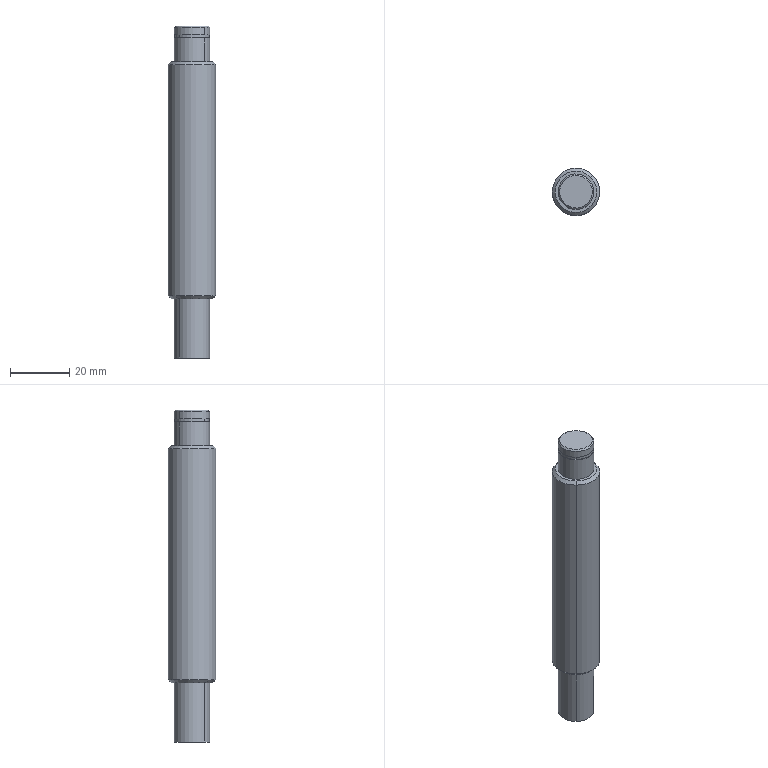Component | SolidWorks | SL010-LeftStreamline-1-1_SL010-2M-0112-000-2-1-1_SL010-LXFB-0102017-1-2 | 1 solid | 22 faces | box 16 x 16 x 112 mm | volume 19641 mm3 | cylinder 10 | cone 6 | plane 6 | commonest cylinder face diameters 12 x6 11.5 x2 16 x2 | material S45C
build123d program:
from build123d import *

# Parameters (mm, degrees)
SKETCH1_W     = 80
SKETCH1_H     = 8
SKETCH3_W     = 1.1
SKETCH3_H     = 16
SKETCH4_W     = 20
SKETCH4_H     = 6
CHAMFER1_SIZE = 1


with BuildPart() as part:
    # Sketch1 → Revolve1 (revolve)
    with BuildSketch(Plane.XY, mode=Mode.PRIVATE) as revolve1_sk:
        with Locations((52, 4)):
            Rectangle(SKETCH1_W, SKETCH1_H)
    revolve(revolve1_sk.sketch.rotate(Axis((92, 0, 0), (-1, 0, 0)), 180), axis=Axis((92, 0, 0), (-1, 0, 0)))

    # Sketch2 → Revolve2 (revolve)
    with BuildSketch(Plane.XY, mode=Mode.PRIVATE) as revolve2_sk:
        Polygon((0, 0), (0, 5.5), (0.5, 6), (12, 6), (12, 0), align=None)
    revolve(revolve2_sk.sketch.rotate(Axis((12, 0, 0), (-1, 0, 0)), 270), axis=Axis((12, 0, 0), (-1, 0, 0)))

    # Sketch3 → Cut-Revolve1 (revolve, cut)
    with BuildSketch(Plane.XY, mode=Mode.PRIVATE) as cut_revolve1_sk:
        with Locations((3.45, 13.75)):
            Rectangle(SKETCH3_W, SKETCH3_H)
    revolve(cut_revolve1_sk.sketch.rotate(Axis((200, 0, 0), (-1, 0, 0)), 270), axis=Axis((200, 0, 0), (-1, 0, 0)), mode=Mode.SUBTRACT)

    # Sketch4 → Revolve3 (revolve)
    with BuildSketch(Plane.XY, mode=Mode.PRIVATE) as revolve3_sk:
        with Locations((102, 3)):
            Rectangle(SKETCH4_W, SKETCH4_H)
    revolve(revolve3_sk.sketch.rotate(Axis((112, 0, 0), (-1, 0, 0)), 180), axis=Axis((112, 0, 0), (-1, 0, 0)))

    # Chamfer1
    chamfer1_edges = [part.edges().sort_by_distance(p)[0] for p in [
        (92, 8, 0),
        (12, 8, 0),
    ]]
    chamfer(chamfer1_edges, length=CHAMFER1_SIZE)


solid = part.part

# Placed as in the assembly
solid = solid.moved(Location((-175, -164.904, -654.035), (0, 90, 0)))
STEP:
#1=COLOUR_RGB('',0.7922,0.8196,0.9333);
#2=FILL_AREA_STYLE_COLOUR('',#1);
#3=FILL_AREA_STYLE('',(#2));
#4=SURFACE_STYLE_FILL_AREA(#3);
#5=SURFACE_SIDE_STYLE('',(#4));
#6=SURFACE_STYLE_USAGE(.BOTH.,#5);
#7=PRESENTATION_STYLE_ASSIGNMENT((#6));
#8=CARTESIAN_POINT('',(-7.085,-6.687,-29.371));
#9=VERTEX_POINT('',#8);
#10=CARTESIAN_POINT('',(-6.695,-6.297,-29.371));
#11=VERTEX_POINT('',#10);
#12=CARTESIAN_POINT('',(-6.89,-6.492,-29.371));
#13=DIRECTION('',(0.,-0.,-1.));
#14=DIRECTION('',(0.7066,0.7076,0.));
#15=AXIS2_PLACEMENT_3D('',#12,#13,#14);
#16=CIRCLE('',#15,0.2756);
#17=EDGE_CURVE('',#9,#11,#16,.T.);
#18=ORIENTED_EDGE('',*,*,#17,.F.);
#19=CARTESIAN_POINT('',(-7.112,-6.715,-29.332));
#20=VERTEX_POINT('',#19);
#21=CARTESIAN_POINT('',(-7.112,-6.715,-29.332));
#22=DIRECTION('',(-0.4997,-0.5003,0.7071));
#23=VECTOR('',#22,39.37);
#24=LINE('',#21,#23);
#25=EDGE_CURVE('',#9,#20,#24,.T.);
#26=ORIENTED_EDGE('',*,*,#25,.T.);
#27=CARTESIAN_POINT('',(-6.667,-6.269,-29.332));
#28=VERTEX_POINT('',#27);
#29=CARTESIAN_POINT('',(-6.89,-6.492,-29.332));
#30=DIRECTION('',(-0.,0.,1.));
#31=DIRECTION('',(0.7066,0.7076,0.));
#32=AXIS2_PLACEMENT_3D('',#29,#30,#31);
#33=CIRCLE('',#32,0.315);
#34=EDGE_CURVE('',#28,#20,#33,.T.);
#35=ORIENTED_EDGE('',*,*,#34,.F.);
#36=CARTESIAN_POINT('',(-6.667,-6.269,-29.332));
#37=DIRECTION('',(0.4997,0.5003,0.7071));
#38=VECTOR('',#37,39.37);
#39=LINE('',#36,#38);
#40=EDGE_CURVE('',#11,#28,#39,.T.);
#41=ORIENTED_EDGE('',*,*,#40,.F.);
#42=EDGE_LOOP('',(#18,#26,#35,#41));
#43=FACE_OUTER_BOUND('',#42,.T.);
#44=CARTESIAN_POINT('',(-6.89,-6.492,-29.332));
#45=DIRECTION('',(-0.,0.,1.));
#46=DIRECTION('',(0.7066,0.7076,0.));
#47=AXIS2_PLACEMENT_3D('',#44,#45,#46);
#48=CONICAL_SURFACE('',#47,0.315,0.7854);
#49=ADVANCED_FACE('',(#43),#48,.T.);
#50=CARTESIAN_POINT('',(-6.695,-6.297,-26.222));
#51=VERTEX_POINT('',#50);
#52=CARTESIAN_POINT('',(-7.085,-6.687,-26.222));
#53=VERTEX_POINT('',#52);
#54=CARTESIAN_POINT('',(-6.89,-6.492,-26.222));
#55=DIRECTION('',(-0.,0.,1.));
#56=DIRECTION('',(-0.7066,-0.7076,0.));
#57=AXIS2_PLACEMENT_3D('',#54,#55,#56);
#58=CIRCLE('',#57,0.2756);
#59=EDGE_CURVE('',#51,#53,#58,.T.);
#60=ORIENTED_EDGE('',*,*,#59,.F.);
#61=CARTESIAN_POINT('',(-6.667,-6.269,-26.261));
#62=VERTEX_POINT('',#61);
#63=CARTESIAN_POINT('',(-6.695,-6.297,-26.222));
#64=DIRECTION('',(0.4997,0.5003,-0.7071));
#65=VECTOR('',#64,39.37);
#66=LINE('',#63,#65);
#67=EDGE_CURVE('',#51,#62,#66,.T.);
#68=ORIENTED_EDGE('',*,*,#67,.T.);
#69=CARTESIAN_POINT('',(-7.112,-6.715,-26.261));
#70=VERTEX_POINT('',#69);
#71=CARTESIAN_POINT('',(-6.89,-6.492,-26.261));
#72=DIRECTION('',(0.,-0.,-1.));
#73=DIRECTION('',(-0.7066,-0.7076,0.));
#74=AXIS2_PLACEMENT_3D('',#71,#72,#73);
#75=CIRCLE('',#74,0.315);
#76=EDGE_CURVE('',#70,#62,#75,.T.);
#77=ORIENTED_EDGE('',*,*,#76,.F.);
#78=CARTESIAN_POINT('',(-7.085,-6.687,-26.222));
#79=DIRECTION('',(-0.4997,-0.5003,-0.7071));
#80=VECTOR('',#79,39.37);
#81=LINE('',#78,#80);
#82=EDGE_CURVE('',#53,#70,#81,.T.);
#83=ORIENTED_EDGE('',*,*,#82,.F.);
#84=EDGE_LOOP('',(#60,#68,#77,#83));
#85=FACE_OUTER_BOUND('',#84,.T.);
#86=CARTESIAN_POINT('',(-6.89,-6.492,-26.222));
#87=DIRECTION('',(0.,-0.,-1.));
#88=DIRECTION('',(-0.7066,-0.7076,0.));
#89=AXIS2_PLACEMENT_3D('',#86,#87,#88);
#90=CONICAL_SURFACE('',#89,0.2756,0.7854);
#91=ADVANCED_FACE('',(#85),#90,.T.);
#92=CARTESIAN_POINT('',(-6.723,-6.325,-30.159));
#93=VERTEX_POINT('',#92);
#94=CARTESIAN_POINT('',(-7.057,-6.659,-30.159));
#95=VERTEX_POINT('',#94);
#96=CARTESIAN_POINT('',(-6.89,-6.492,-30.159));
#97=DIRECTION('',(-0.,0.,1.));
#98=DIRECTION('',(0.7066,0.7076,0.));
#99=AXIS2_PLACEMENT_3D('',#96,#97,#98);
#100=CIRCLE('',#99,0.2362);
#101=EDGE_CURVE('',#93,#95,#100,.T.);
#102=ORIENTED_EDGE('',*,*,#101,.T.);
#103=CARTESIAN_POINT('',(-7.057,-6.659,-29.371));
#104=VERTEX_POINT('',#103);
#105=CARTESIAN_POINT('',(-7.057,-6.659,-30.159));
#106=DIRECTION('',(-0.,0.,1.));
#107=VECTOR('',#106,39.37);
#108=LINE('',#105,#107);
#109=EDGE_CURVE('',#95,#104,#108,.T.);
#110=ORIENTED_EDGE('',*,*,#109,.T.);
#111=CARTESIAN_POINT('',(-6.723,-6.325,-29.371));
#112=VERTEX_POINT('',#111);
#113=CARTESIAN_POINT('',(-6.89,-6.492,-29.371));
#114=DIRECTION('',(0.,-0.,-1.));
#115=DIRECTION('',(0.7066,0.7076,0.));
#116=AXIS2_PLACEMENT_3D('',#113,#114,#115);
#117=CIRCLE('',#116,0.2362);
#118=EDGE_CURVE('',#104,#112,#117,.T.);
#119=ORIENTED_EDGE('',*,*,#118,.T.);
#120=CARTESIAN_POINT('',(-6.723,-6.325,-30.159));
#121=DIRECTION('',(-0.,0.,1.));
#122=VECTOR('',#121,39.37);
#123=LINE('',#120,#122);
#124=EDGE_CURVE('',#93,#112,#123,.T.);
#125=ORIENTED_EDGE('',*,*,#124,.F.);
#126=EDGE_LOOP('',(#102,#110,#119,#125));
#127=FACE_OUTER_BOUND('',#126,.T.);
#128=CARTESIAN_POINT('',(-6.89,-6.492,-30.159));
#129=DIRECTION('',(-0.,0.,1.));
#130=DIRECTION('',(0.7066,0.7076,0.));
#131=AXIS2_PLACEMENT_3D('',#128,#129,#130);
#132=CYLINDRICAL_SURFACE('',#131,0.2362);
#133=ADVANCED_FACE('',(#127),#132,.T.);
#134=CARTESIAN_POINT('',(-6.723,-6.659,-25.864));
#135=VERTEX_POINT('',#134);
#136=CARTESIAN_POINT('',(-7.057,-6.325,-25.864));
#137=VERTEX_POINT('',#136);
#138=CARTESIAN_POINT('',(-6.89,-6.492,-25.864));
#139=DIRECTION('',(-0.,-0.,-1.));
#140=DIRECTION('',(-0.7066,-0.7076,0.));
#141=AXIS2_PLACEMENT_3D('',#138,#139,#140);
#142=CIRCLE('',#141,0.2362);
#143=EDGE_CURVE('',#135,#137,#142,.T.);
#144=ORIENTED_EDGE('',*,*,#143,.F.);
#145=CARTESIAN_POINT('',(-6.723,-6.659,-25.769));
#146=VERTEX_POINT('',#145);
#147=CARTESIAN_POINT('',(-6.723,-6.659,-26.222));
#148=DIRECTION('',(-0.,0.,1.));
#149=VECTOR('',#148,39.37);
#150=LINE('',#147,#149);
#151=EDGE_CURVE('',#135,#146,#150,.T.);
#152=ORIENTED_EDGE('',*,*,#151,.T.);
#153=CARTESIAN_POINT('',(-7.057,-6.325,-25.769));
#154=VERTEX_POINT('',#153);
#155=CARTESIAN_POINT('',(-6.89,-6.492,-25.769));
#156=DIRECTION('',(-0.,0.,1.));
#157=DIRECTION('',(-0.7076,0.7066,0.));
#158=AXIS2_PLACEMENT_3D('',#155,#156,#157);
#159=CIRCLE('',#158,0.2362);
#160=EDGE_CURVE('',#154,#146,#159,.T.);
#161=ORIENTED_EDGE('',*,*,#160,.F.);
#162=CARTESIAN_POINT('',(-7.057,-6.325,-26.222));
#163=DIRECTION('',(-0.,0.,1.));
#164=VECTOR('',#163,39.37);
#165=LINE('',#162,#164);
#166=EDGE_CURVE('',#137,#154,#165,.T.);
#167=ORIENTED_EDGE('',*,*,#166,.F.);
#168=EDGE_LOOP('',(#144,#152,#161,#167));
#169=FACE_OUTER_BOUND('',#168,.T.);
#170=CARTESIAN_POINT('',(-6.89,-6.492,-26.222));
#171=DIRECTION('',(-0.,0.,1.));
#172=DIRECTION('',(-0.7076,0.7066,0.));
#173=AXIS2_PLACEMENT_3D('',#170,#171,#172);
#174=CYLINDRICAL_SURFACE('',#173,0.2362);
#175=ADVANCED_FACE('',(#169),#174,.T.);
#176=CARTESIAN_POINT('',(-7.043,-6.339,-25.749));
#177=VERTEX_POINT('',#176);
#178=CARTESIAN_POINT('',(-6.737,-6.645,-25.749));
#179=VERTEX_POINT('',#178);
#180=CARTESIAN_POINT('',(-6.89,-6.492,-25.749));
#181=DIRECTION('',(-0.,0.,1.));
#182=DIRECTION('',(-0.7076,0.7066,0.));
#183=AXIS2_PLACEMENT_3D('',#180,#181,#182);
#184=CIRCLE('',#183,0.2165);
#185=EDGE_CURVE('',#177,#179,#184,.T.);
#186=ORIENTED_EDGE('',*,*,#185,.F.);
#187=CARTESIAN_POINT('',(-7.057,-6.325,-25.769));
#188=DIRECTION('',(-0.5003,0.4997,-0.7071));
#189=VECTOR('',#188,39.37);
#190=LINE('',#187,#189);
#191=EDGE_CURVE('',#177,#154,#190,.T.);
#192=ORIENTED_EDGE('',*,*,#191,.T.);
#193=ORIENTED_EDGE('',*,*,#160,.T.);
#194=CARTESIAN_POINT('',(-6.723,-6.659,-25.769));
#195=DIRECTION('',(0.5003,-0.4997,-0.7071));
#196=VECTOR('',#195,39.37);
#197=LINE('',#194,#196);
#198=EDGE_CURVE('',#179,#146,#197,.T.);
#199=ORIENTED_EDGE('',*,*,#198,.F.);
#200=EDGE_LOOP('',(#186,#192,#193,#199));
#201=FACE_OUTER_BOUND('',#200,.T.);
#202=CARTESIAN_POINT('',(-6.89,-6.492,-25.769));
#203=DIRECTION('',(0.,-0.,-1.));
#204=DIRECTION('',(0.7076,-0.7066,0.));
#205=AXIS2_PLACEMENT_3D('',#202,#203,#204);
#206=CONICAL_SURFACE('',#205,0.2362,0.7854);
#207=ADVANCED_FACE('',(#201),#206,.T.);
#208=CARTESIAN_POINT('',(-6.73,-6.332,-25.907));
#209=VERTEX_POINT('',#208);
#210=CARTESIAN_POINT('',(-7.05,-6.652,-25.907));
#211=VERTEX_POINT('',#210);
#212=CARTESIAN_POINT('',(-6.89,-6.492,-25.907));
#213=DIRECTION('',(0.,0.,1.));
#214=DIRECTION('',(0.7066,0.7076,0.));
#215=AXIS2_PLACEMENT_3D('',#212,#213,#214);
#216=CIRCLE('',#215,0.2264);
#217=EDGE_CURVE('',#209,#211,#216,.T.);
#218=ORIENTED_EDGE('',*,*,#217,.T.);
#219=CARTESIAN_POINT('',(-7.05,-6.652,-25.864));
#220=VERTEX_POINT('',#219);
#221=CARTESIAN_POINT('',(-7.05,-6.652,-33.623));
#222=DIRECTION('',(0.,0.,1.));
#223=VECTOR('',#222,39.37);
#224=LINE('',#221,#223);
#225=EDGE_CURVE('',#211,#220,#224,.T.);
#226=ORIENTED_EDGE('',*,*,#225,.T.);
#227=CARTESIAN_POINT('',(-6.73,-6.332,-25.864));
#228=VERTEX_POINT('',#227);
#229=CARTESIAN_POINT('',(-6.89,-6.492,-25.864));
#230=DIRECTION('',(0.,0.,1.));
#231=DIRECTION('',(0.7066,0.7076,0.));
#232=AXIS2_PLACEMENT_3D('',#229,#230,#231);
#233=CIRCLE('',#232,0.2264);
#234=EDGE_CURVE('',#228,#220,#233,.T.);
#235=ORIENTED_EDGE('',*,*,#234,.F.);
#236=CARTESIAN_POINT('',(-6.73,-6.332,-33.623));
#237=DIRECTION('',(0.,0.,1.));
#238=VECTOR('',#237,39.37);
#239=LINE('',#236,#238);
#240=EDGE_CURVE('',#209,#228,#239,.T.);
#241=ORIENTED_EDGE('',*,*,#240,.F.);
#242=EDGE_LOOP('',(#218,#226,#235,#241));
#243=FACE_OUTER_BOUND('',#242,.T.);
#244=CARTESIAN_POINT('',(-6.89,-6.492,-33.623));
#245=DIRECTION('',(0.,0.,1.));
#246=DIRECTION('',(0.7066,0.7076,0.));
#247=AXIS2_PLACEMENT_3D('',#244,#245,#246);
#248=CYLINDRICAL_SURFACE('',#247,0.2264);
#249=ADVANCED_FACE('',(#243),#248,.T.);
#250=ORIENTED_EDGE('',*,*,#34,.T.);
#251=CARTESIAN_POINT('',(-7.112,-6.715,-29.371));
#252=DIRECTION('',(-0.,0.,1.));
#253=VECTOR('',#252,39.37);
#254=LINE('',#251,#253);
#255=EDGE_CURVE('',#20,#70,#254,.T.);
#256=ORIENTED_EDGE('',*,*,#255,.T.);
#257=ORIENTED_EDGE('',*,*,#76,.T.);
#258=CARTESIAN_POINT('',(-6.667,-6.269,-29.371));
#259=DIRECTION('',(-0.,0.,1.));
#260=VECTOR('',#259,39.37);
#261=LINE('',#258,#260);
#262=EDGE_CURVE('',#28,#62,#261,.T.);
#263=ORIENTED_EDGE('',*,*,#262,.F.);
#264=EDGE_LOOP('',(#250,#256,#257,#263));
#265=FACE_OUTER_BOUND('',#264,.T.);
#266=CARTESIAN_POINT('',(-6.89,-6.492,-29.371));
#267=DIRECTION('',(-0.,0.,1.));
#268=DIRECTION('',(0.7066,0.7076,0.));
#269=AXIS2_PLACEMENT_3D('',#266,#267,#268);
#270=CYLINDRICAL_SURFACE('',#269,0.315);
#271=ADVANCED_FACE('',(#265),#270,.T.);
#272=CARTESIAN_POINT('',(-7.057,-6.325,-26.222));
#273=VERTEX_POINT('',#272);
#274=CARTESIAN_POINT('',(-6.723,-6.659,-26.222));
#275=VERTEX_POINT('',#274);
#276=CARTESIAN_POINT('',(-6.89,-6.492,-26.222));
#277=DIRECTION('',(-0.,0.,1.));
#278=DIRECTION('',(-0.7066,-0.7076,0.));
#279=AXIS2_PLACEMENT_3D('',#276,#277,#278);
#280=CIRCLE('',#279,0.2362);
#281=EDGE_CURVE('',#273,#275,#280,.T.);
#282=ORIENTED_EDGE('',*,*,#281,.T.);
#283=CARTESIAN_POINT('',(-6.723,-6.659,-25.907));
#284=VERTEX_POINT('',#283);
#285=CARTESIAN_POINT('',(-6.723,-6.659,-26.222));
#286=DIRECTION('',(-0.,0.,1.));
#287=VECTOR('',#286,39.37);
#288=LINE('',#285,#287);
#289=EDGE_CURVE('',#275,#284,#288,.T.);
#290=ORIENTED_EDGE('',*,*,#289,.T.);
#291=CARTESIAN_POINT('',(-7.057,-6.325,-25.907));
#292=VERTEX_POINT('',#291);
#293=CARTESIAN_POINT('',(-6.89,-6.492,-25.907));
#294=DIRECTION('',(0.,0.,1.));
#295=DIRECTION('',(0.7066,0.7076,0.));
#296=AXIS2_PLACEMENT_3D('',#293,#294,#295);
#297=CIRCLE('',#296,0.2362);
#298=EDGE_CURVE('',#292,#284,#297,.T.);
#299=ORIENTED_EDGE('',*,*,#298,.F.);
#300=CARTESIAN_POINT('',(-7.057,-6.325,-26.222));
#301=DIRECTION('',(-0.,0.,1.));
#302=VECTOR('',#301,39.37);
#303=LINE('',#300,#302);
#304=EDGE_CURVE('',#273,#292,#303,.T.);
#305=ORIENTED_EDGE('',*,*,#304,.F.);
#306=EDGE_LOOP('',(#282,#290,#299,#305));
#307=FACE_OUTER_BOUND('',#306,.T.);
#308=CARTESIAN_POINT('',(-6.89,-6.492,-26.222));
#309=DIRECTION('',(-0.,0.,1.));
#310=DIRECTION('',(-0.7076,0.7066,0.));
#311=AXIS2_PLACEMENT_3D('',#308,#309,#310);
#312=CYLINDRICAL_SURFACE('',#311,0.2362);
#313=ADVANCED_FACE('',(#307),#312,.T.);
#314=CARTESIAN_POINT('',(-6.89,-6.492,-29.371));
#315=DIRECTION('',(0.,-0.,-1.));
#316=DIRECTION('',(0.7066,0.7076,0.));
#317=AXIS2_PLACEMENT_3D('',#314,#315,#316);
#318=CIRCLE('',#317,0.2756);
#319=EDGE_CURVE('',#11,#9,#318,.T.);
#320=ORIENTED_EDGE('',*,*,#319,.T.);
#321=ORIENTED_EDGE('',*,*,#17,.T.);
#322=EDGE_LOOP('',(#320,#321));
#323=FACE_OUTER_BOUND('',#322,.T.);
#324=CARTESIAN_POINT('',(-6.89,-6.492,-29.371));
#325=DIRECTION('',(0.,-0.,-1.));
#326=DIRECTION('',(0.7066,0.7076,0.));
#327=AXIS2_PLACEMENT_3D('',#324,#325,#326);
#328=CIRCLE('',#327,0.2362);
#329=EDGE_CURVE('',#112,#104,#328,.T.);
#330=ORIENTED_EDGE('',*,*,#329,.F.);
#331=ORIENTED_EDGE('',*,*,#118,.F.);
#332=EDGE_LOOP('',(#330,#331));
#333=FACE_BOUND('',#332,.T.);
#334=CARTESIAN_POINT('',(-7.112,-6.715,-29.371));
#335=DIRECTION('',(-0.,0.,1.));
#336=DIRECTION('',(0.7066,0.7076,-0.));
#337=AXIS2_PLACEMENT_3D('',#334,#335,#336);
#338=PLANE('',#337);
#339=ADVANCED_FACE('',(#323,#333),#338,.F.);
#340=ORIENTED_EDGE('',*,*,#289,.F.);
#341=CARTESIAN_POINT('',(-6.89,-6.492,-26.222));
#342=DIRECTION('',(-0.,0.,1.));
#343=DIRECTION('',(-0.7066,-0.7076,0.));
#344=AXIS2_PLACEMENT_3D('',#341,#342,#343);
#345=CIRCLE('',#344,0.2362);
#346=EDGE_CURVE('',#275,#273,#345,.T.);
#347=ORIENTED_EDGE('',*,*,#346,.T.);
#348=ORIENTED_EDGE('',*,*,#304,.T.);
#349=CARTESIAN_POINT('',(-6.89,-6.492,-25.907));
#350=DIRECTION('',(0.,0.,1.));
#351=DIRECTION('',(0.7066,0.7076,0.));
#352=AXIS2_PLACEMENT_3D('',#349,#350,#351);
#353=CIRCLE('',#352,0.2362);
#354=EDGE_CURVE('',#284,#292,#353,.T.);
#355=ORIENTED_EDGE('',*,*,#354,.F.);
#356=EDGE_LOOP('',(#340,#347,#348,#355));
#357=FACE_OUTER_BOUND('',#356,.T.);
#358=CARTESIAN_POINT('',(-6.89,-6.492,-26.222));
#359=DIRECTION('',(-0.,0.,1.));
#360=DIRECTION('',(-0.7076,0.7066,0.));
#361=AXIS2_PLACEMENT_3D('',#358,#359,#360);
#362=CYLINDRICAL_SURFACE('',#361,0.2362);
#363=ADVANCED_FACE('',(#357),#362,.T.);
#364=CARTESIAN_POINT('',(-6.89,-6.492,-26.222));
#365=DIRECTION('',(-0.,0.,1.));
#366=DIRECTION('',(-0.7066,-0.7076,0.));
#367=AXIS2_PLACEMENT_3D('',#364,#365,#366);
#368=CIRCLE('',#367,0.2756);
#369=EDGE_CURVE('',#53,#51,#368,.T.);
#370=ORIENTED_EDGE('',*,*,#369,.T.);
#371=ORIENTED_EDGE('',*,*,#59,.T.);
#372=EDGE_LOOP('',(#370,#371));
#373=FACE_OUTER_BOUND('',#372,.T.);
#374=ORIENTED_EDGE('',*,*,#281,.F.);
#375=ORIENTED_EDGE('',*,*,#346,.F.);
#376=EDGE_LOOP('',(#374,#375));
#377=FACE_BOUND('',#376,.T.);
#378=CARTESIAN_POINT('',(-6.89,-6.492,-26.222));
#379=DIRECTION('',(0.,-0.,-1.));
#380=DIRECTION('',(-0.7066,-0.7076,0.));
#381=AXIS2_PLACEMENT_3D('',#378,#379,#380);
#382=PLANE('',#381);
#383=ADVANCED_FACE('',(#373,#377),#382,.F.);
#384=ORIENTED_EDGE('',*,*,#255,.F.);
#385=CARTESIAN_POINT('',(-6.89,-6.492,-29.332));
#386=DIRECTION('',(-0.,0.,1.));
#387=DIRECTION('',(0.7066,0.7076,0.));
#388=AXIS2_PLACEMENT_3D('',#385,#386,#387);
#389=CIRCLE('',#388,0.315);
#390=EDGE_CURVE('',#20,#28,#389,.T.);
#391=ORIENTED_EDGE('',*,*,#390,.T.);
#392=ORIENTED_EDGE('',*,*,#262,.T.);
#393=CARTESIAN_POINT('',(-6.89,-6.492,-26.261));
#394=DIRECTION('',(0.,-0.,-1.));
#395=DIRECTION('',(-0.7066,-0.7076,0.));
#396=AXIS2_PLACEMENT_3D('',#393,#394,#395);
#397=CIRCLE('',#396,0.315);
#398=EDGE_CURVE('',#62,#70,#397,.T.);
#399=ORIENTED_EDGE('',*,*,#398,.T.);
#400=EDGE_LOOP('',(#384,#391,#392,#399));
#401=FACE_OUTER_BOUND('',#400,.T.);
#402=CARTESIAN_POINT('',(-6.89,-6.492,-29.371));
#403=DIRECTION('',(-0.,0.,1.));
#404=DIRECTION('',(0.7066,0.7076,0.));
#405=AXIS2_PLACEMENT_3D('',#402,#403,#404);
#406=CYLINDRICAL_SURFACE('',#405,0.315);
#407=ADVANCED_FACE('',(#401),#406,.T.);
#408=ORIENTED_EDGE('',*,*,#234,.T.);
#409=CARTESIAN_POINT('',(-6.89,-6.492,-25.864));
#410=DIRECTION('',(0.,0.,1.));
#411=DIRECTION('',(0.7066,0.7076,0.));
#412=AXIS2_PLACEMENT_3D('',#409,#410,#411);
#413=CIRCLE('',#412,0.2264);
#414=EDGE_CURVE('',#220,#228,#413,.T.);
#415=ORIENTED_EDGE('',*,*,#414,.T.);
#416=EDGE_LOOP('',(#408,#415));
#417=FACE_BOUND('',#416,.T.);
#418=CARTESIAN_POINT('',(-6.89,-6.492,-25.864));
#419=DIRECTION('',(-0.,-0.,-1.));
#420=DIRECTION('',(-0.7066,-0.7076,0.));
#421=AXIS2_PLACEMENT_3D('',#418,#419,#420);
#422=CIRCLE('',#421,0.2362);
#423=EDGE_CURVE('',#137,#135,#422,.T.);
#424=ORIENTED_EDGE('',*,*,#423,.T.);
#425=ORIENTED_EDGE('',*,*,#143,.T.);
#426=EDGE_LOOP('',(#424,#425));
#427=FACE_OUTER_BOUND('',#426,.T.);
#428=CARTESIAN_POINT('',(-7.495,-7.098,-25.864));
#429=DIRECTION('',(-0.,-0.,-1.));
#430=DIRECTION('',(-0.7066,-0.7076,0.));
#431=AXIS2_PLACEMENT_3D('',#428,#429,#430);
#432=PLANE('',#431);
#433=ADVANCED_FACE('',(#417,#427),#432,.T.);
#434=ORIENTED_EDGE('',*,*,#217,.F.);
#435=CARTESIAN_POINT('',(-6.89,-6.492,-25.907));
#436=DIRECTION('',(0.,0.,1.));
#437=DIRECTION('',(0.7066,0.7076,0.));
#438=AXIS2_PLACEMENT_3D('',#435,#436,#437);
#439=CIRCLE('',#438,0.2264);
#440=EDGE_CURVE('',#211,#209,#439,.T.);
#441=ORIENTED_EDGE('',*,*,#440,.F.);
#442=EDGE_LOOP('',(#434,#441));
#443=FACE_BOUND('',#442,.T.);
#444=ORIENTED_EDGE('',*,*,#298,.T.);
#445=ORIENTED_EDGE('',*,*,#354,.T.);
#446=EDGE_LOOP('',(#444,#445));
#447=FACE_OUTER_BOUND('',#446,.T.);
#448=CARTESIAN_POINT('',(-7.05,-6.652,-25.907));
#449=DIRECTION('',(0.,0.,1.));
#450=DIRECTION('',(0.7066,0.7076,-0.));
#451=AXIS2_PLACEMENT_3D('',#448,#449,#450);
#452=PLANE('',#451);
#453=ADVANCED_FACE('',(#443,#447),#452,.T.);
#454=ORIENTED_EDGE('',*,*,#225,.F.);
#455=ORIENTED_EDGE('',*,*,#440,.T.);
#456=ORIENTED_EDGE('',*,*,#240,.T.);
#457=ORIENTED_EDGE('',*,*,#414,.F.);
#458=EDGE_LOOP('',(#454,#455,#456,#457));
#459=FACE_OUTER_BOUND('',#458,.T.);
#460=CARTESIAN_POINT('',(-6.89,-6.492,-33.623));
#461=DIRECTION('',(0.,0.,1.));
#462=DIRECTION('',(0.7066,0.7076,0.));
#463=AXIS2_PLACEMENT_3D('',#460,#461,#462);
#464=CYLINDRICAL_SURFACE('',#463,0.2264);
#465=ADVANCED_FACE('',(#459),#464,.T.);
#466=CARTESIAN_POINT('',(-6.89,-6.492,-25.749));
#467=DIRECTION('',(-0.,0.,1.));
#468=DIRECTION('',(-0.7076,0.7066,0.));
#469=AXIS2_PLACEMENT_3D('',#466,#467,#468);
#470=CIRCLE('',#469,0.2165);
#471=EDGE_CURVE('',#179,#177,#470,.T.);
#472=ORIENTED_EDGE('',*,*,#471,.T.);
#473=ORIENTED_EDGE('',*,*,#185,.T.);
#474=EDGE_LOOP('',(#472,#473));
#475=FACE_OUTER_BOUND('',#474,.T.);
#476=CARTESIAN_POINT('',(-6.89,-6.492,-25.749));
#477=DIRECTION('',(0.,-0.,-1.));
#478=DIRECTION('',(0.7076,-0.7066,0.));
#479=AXIS2_PLACEMENT_3D('',#476,#477,#478);
#480=PLANE('',#479);
#481=ADVANCED_FACE('',(#475),#480,.F.);
#482=ORIENTED_EDGE('',*,*,#191,.F.);
#483=ORIENTED_EDGE('',*,*,#471,.F.);
#484=ORIENTED_EDGE('',*,*,#198,.T.);
#485=CARTESIAN_POINT('',(-6.89,-6.492,-25.769));
#486=DIRECTION('',(-0.,0.,1.));
#487=DIRECTION('',(-0.7076,0.7066,0.));
#488=AXIS2_PLACEMENT_3D('',#485,#486,#487);
#489=CIRCLE('',#488,0.2362);
#490=EDGE_CURVE('',#146,#154,#489,.T.);
#491=ORIENTED_EDGE('',*,*,#490,.T.);
#492=EDGE_LOOP('',(#482,#483,#484,#491));
#493=FACE_OUTER_BOUND('',#492,.T.);
#494=CARTESIAN_POINT('',(-6.89,-6.492,-25.769));
#495=DIRECTION('',(0.,-0.,-1.));
#496=DIRECTION('',(0.7076,-0.7066,0.));
#497=AXIS2_PLACEMENT_3D('',#494,#495,#496);
#498=CONICAL_SURFACE('',#497,0.2362,0.7854);
#499=ADVANCED_FACE('',(#493),#498,.T.);
#500=ORIENTED_EDGE('',*,*,#151,.F.);
#501=ORIENTED_EDGE('',*,*,#423,.F.);
#502=ORIENTED_EDGE('',*,*,#166,.T.);
#503=ORIENTED_EDGE('',*,*,#490,.F.);
#504=EDGE_LOOP('',(#500,#501,#502,#503));
#505=FACE_OUTER_BOUND('',#504,.T.);
#506=CARTESIAN_POINT('',(-6.89,-6.492,-26.222));
#507=DIRECTION('',(-0.,0.,1.));
#508=DIRECTION('',(-0.7076,0.7066,0.));
#509=AXIS2_PLACEMENT_3D('',#506,#507,#508);
#510=CYLINDRICAL_SURFACE('',#509,0.2362);
#511=ADVANCED_FACE('',(#505),#510,.T.);
#512=ORIENTED_EDGE('',*,*,#109,.F.);
#513=CARTESIAN_POINT('',(-6.89,-6.492,-30.159));
#514=DIRECTION('',(-0.,0.,1.));
#515=DIRECTION('',(0.7066,0.7076,0.));
#516=AXIS2_PLACEMENT_3D('',#513,#514,#515);
#517=CIRCLE('',#516,0.2362);
#518=EDGE_CURVE('',#95,#93,#517,.T.);
#519=ORIENTED_EDGE('',*,*,#518,.T.);
#520=ORIENTED_EDGE('',*,*,#124,.T.);
#521=ORIENTED_EDGE('',*,*,#329,.T.);
#522=EDGE_LOOP('',(#512,#519,#520,#521));
#523=FACE_OUTER_BOUND('',#522,.T.);
#524=CARTESIAN_POINT('',(-6.89,-6.492,-30.159));
#525=DIRECTION('',(-0.,0.,1.));
#526=DIRECTION('',(0.7066,0.7076,0.));
#527=AXIS2_PLACEMENT_3D('',#524,#525,#526);
#528=CYLINDRICAL_SURFACE('',#527,0.2362);
#529=ADVANCED_FACE('',(#523),#528,.T.);
#530=ORIENTED_EDGE('',*,*,#101,.F.);
#531=ORIENTED_EDGE('',*,*,#518,.F.);
#532=EDGE_LOOP('',(#530,#531));
#533=FACE_OUTER_BOUND('',#532,.T.);
#534=CARTESIAN_POINT('',(-7.057,-6.659,-30.159));
#535=DIRECTION('',(0.,0.,1.));
#536=DIRECTION('',(0.7066,0.7076,-0.));
#537=AXIS2_PLACEMENT_3D('',#534,#535,#536);
#538=PLANE('',#537);
#539=ADVANCED_FACE('',(#533),#538,.F.);
#540=ORIENTED_EDGE('',*,*,#67,.F.);
#541=ORIENTED_EDGE('',*,*,#369,.F.);
#542=ORIENTED_EDGE('',*,*,#82,.T.);
#543=ORIENTED_EDGE('',*,*,#398,.F.);
#544=EDGE_LOOP('',(#540,#541,#542,#543));
#545=FACE_OUTER_BOUND('',#544,.T.);
#546=CARTESIAN_POINT('',(-6.89,-6.492,-26.222));
#547=DIRECTION('',(0.,-0.,-1.));
#548=DIRECTION('',(-0.7066,-0.7076,0.));
#549=AXIS2_PLACEMENT_3D('',#546,#547,#548);
#550=CONICAL_SURFACE('',#549,0.2756,0.7854);
#551=ADVANCED_FACE('',(#545),#550,.T.);
#552=ORIENTED_EDGE('',*,*,#25,.F.);
#553=ORIENTED_EDGE('',*,*,#319,.F.);
#554=ORIENTED_EDGE('',*,*,#40,.T.);
#555=ORIENTED_EDGE('',*,*,#390,.F.);
#556=EDGE_LOOP('',(#552,#553,#554,#555));
#557=FACE_OUTER_BOUND('',#556,.T.);
#558=CARTESIAN_POINT('',(-6.89,-6.492,-29.332));
#559=DIRECTION('',(-0.,0.,1.));
#560=DIRECTION('',(0.7066,0.7076,0.));
#561=AXIS2_PLACEMENT_3D('',#558,#559,#560);
#562=CONICAL_SURFACE('',#561,0.315,0.7854);
#563=ADVANCED_FACE('',(#557),#562,.T.);
#564=CLOSED_SHELL('',(#49,#91,#133,#175,#207,#249,#271,#313,#339,#363,#383,#407,#433,#453,#465,#481,#499,#511,#529,#539,#551,#563));
#565=MANIFOLD_SOLID_BREP('',#564);
#566=STYLED_ITEM('',(#7),#565);
#567=(LENGTH_UNIT()NAMED_UNIT(*)SI_UNIT($,.METRE.));
#568=LENGTH_MEASURE_WITH_UNIT(LENGTH_MEASURE(0.0254),#567);
#569=DIMENSIONAL_EXPONENTS(1.,0.,0.,0.,0.,0.,0.);
#570=(CONVERSION_BASED_UNIT('',#568)LENGTH_UNIT()NAMED_UNIT(#569));
#571=UNCERTAINTY_MEASURE_WITH_UNIT(LENGTH_MEASURE(0.00001),#570,'','');
#572=(NAMED_UNIT(*)PLANE_ANGLE_UNIT()SI_UNIT($,.RADIAN.));
#573=(NAMED_UNIT(*)SI_UNIT($,.STERADIAN.)SOLID_ANGLE_UNIT());
#574=(GEOMETRIC_REPRESENTATION_CONTEXT(3)GLOBAL_UNCERTAINTY_ASSIGNED_CONTEXT((#571))GLOBAL_UNIT_ASSIGNED_CONTEXT((#570,#572,#573))REPRESENTATION_CONTEXT('',''));
#575=MECHANICAL_DESIGN_GEOMETRIC_PRESENTATION_REPRESENTATION('',(#566),#574);
#576=CARTESIAN_POINT('',(0.,0.,0.));
#577=DIRECTION('',(0.,0.,1.));
#578=DIRECTION('',(1.,0.,0.));
#579=AXIS2_PLACEMENT_3D('',#576,#577,#578);
#580=(LENGTH_UNIT()NAMED_UNIT(*)SI_UNIT($,.METRE.));
#581=LENGTH_MEASURE_WITH_UNIT(LENGTH_MEASURE(0.0254),#580);
#582=DIMENSIONAL_EXPONENTS(1.,0.,0.,0.,0.,0.,0.);
#583=(CONVERSION_BASED_UNIT('',#581)LENGTH_UNIT()NAMED_UNIT(#582));
#584=UNCERTAINTY_MEASURE_WITH_UNIT(LENGTH_MEASURE(0.00001),#583,'','');
#585=(NAMED_UNIT(*)PLANE_ANGLE_UNIT()SI_UNIT($,.RADIAN.));
#586=(NAMED_UNIT(*)SI_UNIT($,.STERADIAN.)SOLID_ANGLE_UNIT());
#587=(GEOMETRIC_REPRESENTATION_CONTEXT(3)GLOBAL_UNCERTAINTY_ASSIGNED_CONTEXT((#584))GLOBAL_UNIT_ASSIGNED_CONTEXT((#583,#585,#586))REPRESENTATION_CONTEXT('',''));
#588=ADVANCED_BREP_SHAPE_REPRESENTATION('',(#565,#579),#587);
#589=PRESENTATION_LAYER_ASSIGNMENT('','',(#566));